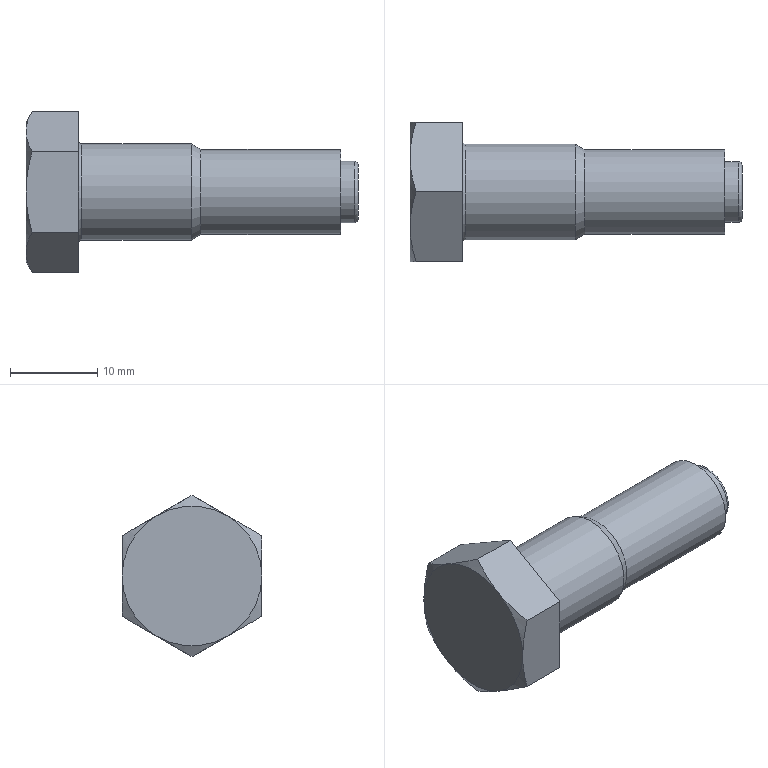Component | NX | GB27-88_M10X32 | 1 solid | 22 faces | volume 3912 mm3 | plane 10 | cone 7 | cylinder 3 | torus 2 | commonest cylinder face diameters 11 x1 9.732 x1 7 x1